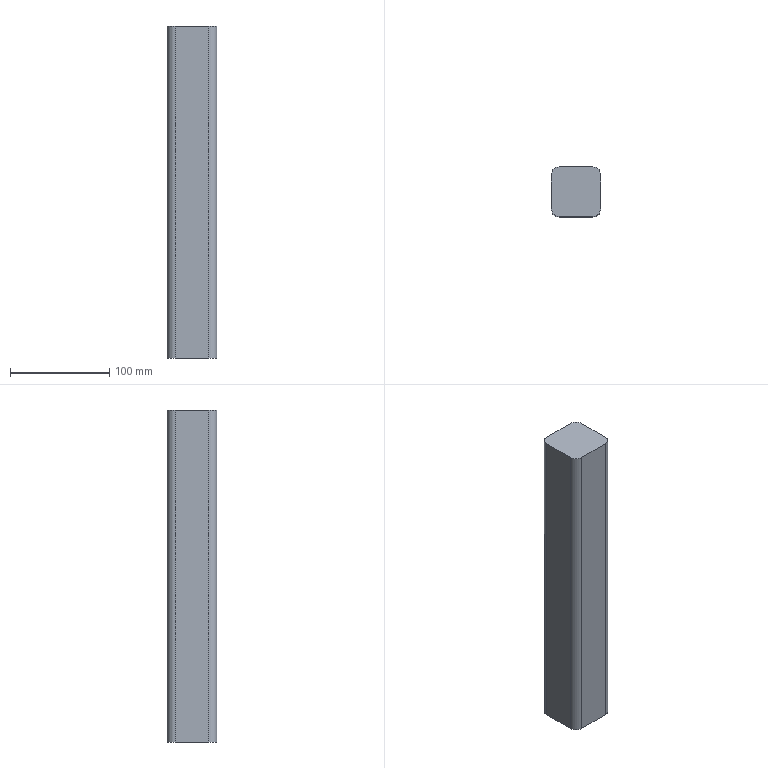Component | SolidWorks | AX00-100.1.1-1_AXFrame_A.1.1-1_AX50x50-5_square tube.1.1-2 | 1 solid | 20 faces | box 50 x 50 x 335 mm | volume 301607 mm3 | plane 12 | cylinder 8 | commonest cylinder face diameters 16 x4 6 x4 | material AISI 1035 Steel (SS)
build123d program:
from build123d import *

# Parameters (mm, degrees)
SKETCH1_W           = 50
SKETCH1_H           = 50
BOSS_EXTRUDE1_DEPTH = 167.5
FILLET3_R           = 8
SHELL1_T            = 5


with BuildPart() as part:
    # Sketch1 → Boss-Extrude1 (new, symmetric)
    with BuildSketch(Plane.XY):
        Rectangle(SKETCH1_W, SKETCH1_H)
    extrude(amount=BOSS_EXTRUDE1_DEPTH, both=True)

    # Fillet3
    fillet3_edges = [part.edges().sort_by_distance(p)[0] for p in [
        (25, -25, 0),
        (-25, -25, 0),
        (-25, 25, 0),
        (25, 25, 0),
    ]]
    fillet(fillet3_edges, radius=FILLET3_R)

    # Shell1 (no face opened: a closed hollow body)
    add(offset(amount=-SHELL1_T, mode=Mode.PRIVATE), mode=Mode.SUBTRACT)


solid = part.part

# Placed as in the assembly
solid = solid.moved(Location((573.631, 1123.364, -5), (0, 0, 0)))